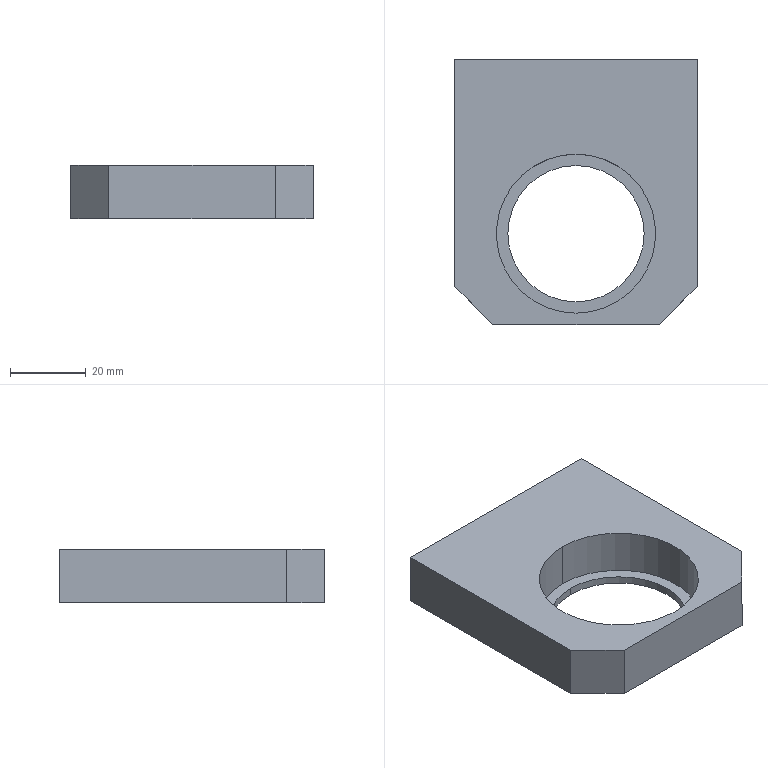Component | SolidWorks | 8TC-A15004-D0-07A-1 | 1 solid | 21 faces | box 64 x 70 x 14 mm | volume 42050 mm3 | plane 9 | cylinder 8 | cone 4 | commonest cylinder face diameters 5 x4 42 x2 36 x2 | material #45
build123d program:
from build123d import *

# Parameters (mm, degrees)
SKETCH1_W             = 64
SKETCH1_H             = 70
BOSS_EXTRUDE1_DEPTH   = 7
SKETCH2_R             = 18
CUT_EXTRUDE1_DEPTH    = 50.447
SKETCH3_R             = 21
CUT_EXTRUDE2_DEPTH    = 12
CHAMFER1_SIZE         = 10
M6_TAPPED_HOLE1_D     = 5
M6_TAPPED_HOLE1_DEPTH = 15
M6_TAPPED_HOLE1_TIP   = 1.502


with BuildPart() as part:
    # Sketch1 → Boss-Extrude1 (new, symmetric)
    with BuildSketch(Plane(origin=(0, 0, 0), x_dir=(1, 0, 0), z_dir=(0, 1, 0))):
        Rectangle(SKETCH1_W, SKETCH1_H)
    extrude(amount=BOSS_EXTRUDE1_DEPTH, both=True)

    # Sketch2 → Cut-Extrude1 (cut, through all)
    with BuildSketch(Plane(origin=(0, 7, 0), x_dir=(1, 0, 0), z_dir=(0, 1, 0))):
        with Locations(Location((0, -11, 0), (0, 0, 270))):
            Circle(SKETCH2_R)
    extrude(amount=-CUT_EXTRUDE1_DEPTH, mode=Mode.SUBTRACT)

    # Sketch3 → Cut-Extrude2 (cut)
    with BuildSketch(Plane(origin=(0, 7, 0), x_dir=(1, 0, 0), z_dir=(0, 1, 0))):
        with Locations(Location((0, -11, 0), (0, 0, 270))):
            Circle(SKETCH3_R)
    extrude(amount=-CUT_EXTRUDE2_DEPTH, mode=Mode.SUBTRACT)

    # Chamfer1
    chamfer1_edges = [part.edges().sort_by_distance(p)[0] for p in [
        (32, 0, 35),
        (-32, 0, 35),
    ]]
    chamfer(chamfer1_edges, length=CHAMFER1_SIZE)

    # M6 Tapped Hole1
    with Locations(Plane(origin=(0, 0, -35), x_dir=(-1, 0, 0), z_dir=(0, 0, -1))):
        with Locations((-25, 0), (25, 0)):
            Hole(M6_TAPPED_HOLE1_D / 2, depth=M6_TAPPED_HOLE1_DEPTH)
            with Locations((0, 0, -(M6_TAPPED_HOLE1_DEPTH + M6_TAPPED_HOLE1_TIP / 2))):  # 118° drill point
                Cone(0, M6_TAPPED_HOLE1_D / 2, M6_TAPPED_HOLE1_TIP, mode=Mode.SUBTRACT)


solid = part.part

# Placed as in the assembly
solid = solid.moved(Location((-7.5, 297.5, -101), (90, 0, 0)))
STEP:
#1=COLOUR_RGB('',0.7922,0.8196,0.9333);
#2=FILL_AREA_STYLE_COLOUR('',#1);
#3=FILL_AREA_STYLE('',(#2));
#4=SURFACE_STYLE_FILL_AREA(#3);
#5=SURFACE_SIDE_STYLE('',(#4));
#6=SURFACE_STYLE_USAGE(.BOTH.,#5);
#7=PRESENTATION_STYLE_ASSIGNMENT((#6));
#8=CARTESIAN_POINT('',(0.7874,12.5,-3.976));
#9=VERTEX_POINT('',#8);
#10=CARTESIAN_POINT('',(0.5906,12.5,-3.976));
#11=VERTEX_POINT('',#10);
#12=CARTESIAN_POINT('',(0.689,12.5,-3.976));
#13=DIRECTION('',(-0.,1.,-0.));
#14=DIRECTION('',(-1.,0.,0.));
#15=AXIS2_PLACEMENT_3D('',#12,#13,#14);
#16=CIRCLE('',#15,0.09843);
#17=EDGE_CURVE('',#9,#11,#16,.T.);
#18=ORIENTED_EDGE('',*,*,#17,.F.);
#19=CARTESIAN_POINT('',(0.7874,13.091,-3.976));
#20=VERTEX_POINT('',#19);
#21=CARTESIAN_POINT('',(0.7874,13.091,-3.976));
#22=DIRECTION('',(-0.,1.,-0.));
#23=VECTOR('',#22,39.37);
#24=LINE('',#21,#23);
#25=EDGE_CURVE('',#9,#20,#24,.T.);
#26=ORIENTED_EDGE('',*,*,#25,.T.);
#27=CARTESIAN_POINT('',(0.5906,13.091,-3.976));
#28=VERTEX_POINT('',#27);
#29=CARTESIAN_POINT('',(0.689,13.091,-3.976));
#30=DIRECTION('',(-0.,1.,-0.));
#31=DIRECTION('',(-1.,0.,0.));
#32=AXIS2_PLACEMENT_3D('',#29,#30,#31);
#33=CIRCLE('',#32,0.09843);
#34=EDGE_CURVE('',#20,#28,#33,.T.);
#35=ORIENTED_EDGE('',*,*,#34,.T.);
#36=CARTESIAN_POINT('',(0.5906,13.091,-3.976));
#37=DIRECTION('',(-0.,1.,-0.));
#38=VECTOR('',#37,39.37);
#39=LINE('',#36,#38);
#40=EDGE_CURVE('',#11,#28,#39,.T.);
#41=ORIENTED_EDGE('',*,*,#40,.F.);
#42=EDGE_LOOP('',(#18,#26,#35,#41));
#43=FACE_OUTER_BOUND('',#42,.T.);
#44=CARTESIAN_POINT('',(0.689,13.091,-3.976));
#45=DIRECTION('',(-0.,1.,-0.));
#46=DIRECTION('',(-1.,0.,0.));
#47=AXIS2_PLACEMENT_3D('',#44,#45,#46);
#48=CYLINDRICAL_SURFACE('',#47,0.09843);
#49=ADVANCED_FACE('',(#43),#48,.F.);
#50=CARTESIAN_POINT('',(0.689,12.441,-3.976));
#51=VERTEX_POINT('',#50);
#52=CARTESIAN_POINT('',(0.5906,12.5,-3.976));
#53=DIRECTION('',(-0.8572,0.515,0.));
#54=VECTOR('',#53,39.37);
#55=LINE('',#52,#54);
#56=EDGE_CURVE('',#51,#11,#55,.T.);
#57=ORIENTED_EDGE('',*,*,#56,.F.);
#58=CARTESIAN_POINT('',(0.7874,12.5,-3.976));
#59=DIRECTION('',(0.8572,0.515,-0.));
#60=VECTOR('',#59,39.37);
#61=LINE('',#58,#60);
#62=EDGE_CURVE('',#51,#9,#61,.T.);
#63=ORIENTED_EDGE('',*,*,#62,.T.);
#64=ORIENTED_EDGE('',*,*,#17,.T.);
#65=EDGE_LOOP('',(#57,#63,#64));
#66=FACE_OUTER_BOUND('',#65,.T.);
#67=CARTESIAN_POINT('',(0.689,12.5,-3.976));
#68=DIRECTION('',(-0.,1.,-0.));
#69=DIRECTION('',(-1.,0.,0.));
#70=AXIS2_PLACEMENT_3D('',#67,#68,#69);
#71=CONICAL_SURFACE('',#70,0.09843,1.03);
#72=ADVANCED_FACE('',(#66),#71,.F.);
#73=CARTESIAN_POINT('',(-1.181,12.5,-3.976));
#74=VERTEX_POINT('',#73);
#75=CARTESIAN_POINT('',(-1.378,12.5,-3.976));
#76=VERTEX_POINT('',#75);
#77=CARTESIAN_POINT('',(-1.28,12.5,-3.976));
#78=DIRECTION('',(-0.,1.,-0.));
#79=DIRECTION('',(-1.,0.,0.));
#80=AXIS2_PLACEMENT_3D('',#77,#78,#79);
#81=CIRCLE('',#80,0.09843);
#82=EDGE_CURVE('',#74,#76,#81,.T.);
#83=ORIENTED_EDGE('',*,*,#82,.F.);
#84=CARTESIAN_POINT('',(-1.181,13.091,-3.976));
#85=VERTEX_POINT('',#84);
#86=CARTESIAN_POINT('',(-1.181,13.091,-3.976));
#87=DIRECTION('',(-0.,1.,-0.));
#88=VECTOR('',#87,39.37);
#89=LINE('',#86,#88);
#90=EDGE_CURVE('',#74,#85,#89,.T.);
#91=ORIENTED_EDGE('',*,*,#90,.T.);
#92=CARTESIAN_POINT('',(-1.378,13.091,-3.976));
#93=VERTEX_POINT('',#92);
#94=CARTESIAN_POINT('',(-1.28,13.091,-3.976));
#95=DIRECTION('',(-0.,1.,-0.));
#96=DIRECTION('',(-1.,0.,0.));
#97=AXIS2_PLACEMENT_3D('',#94,#95,#96);
#98=CIRCLE('',#97,0.09843);
#99=EDGE_CURVE('',#85,#93,#98,.T.);
#100=ORIENTED_EDGE('',*,*,#99,.T.);
#101=CARTESIAN_POINT('',(-1.378,13.091,-3.976));
#102=DIRECTION('',(-0.,1.,-0.));
#103=VECTOR('',#102,39.37);
#104=LINE('',#101,#103);
#105=EDGE_CURVE('',#76,#93,#104,.T.);
#106=ORIENTED_EDGE('',*,*,#105,.F.);
#107=EDGE_LOOP('',(#83,#91,#100,#106));
#108=FACE_OUTER_BOUND('',#107,.T.);
#109=CARTESIAN_POINT('',(-1.28,13.091,-3.976));
#110=DIRECTION('',(-0.,1.,-0.));
#111=DIRECTION('',(-1.,0.,0.));
#112=AXIS2_PLACEMENT_3D('',#109,#110,#111);
#113=CYLINDRICAL_SURFACE('',#112,0.09843);
#114=ADVANCED_FACE('',(#108),#113,.F.);
#115=CARTESIAN_POINT('',(-1.28,12.441,-3.976));
#116=VERTEX_POINT('',#115);
#117=CARTESIAN_POINT('',(-1.378,12.5,-3.976));
#118=DIRECTION('',(-0.8572,0.515,0.));
#119=VECTOR('',#118,39.37);
#120=LINE('',#117,#119);
#121=EDGE_CURVE('',#116,#76,#120,.T.);
#122=ORIENTED_EDGE('',*,*,#121,.F.);
#123=CARTESIAN_POINT('',(-1.181,12.5,-3.976));
#124=DIRECTION('',(0.8572,0.515,-0.));
#125=VECTOR('',#124,39.37);
#126=LINE('',#123,#125);
#127=EDGE_CURVE('',#116,#74,#126,.T.);
#128=ORIENTED_EDGE('',*,*,#127,.T.);
#129=ORIENTED_EDGE('',*,*,#82,.T.);
#130=EDGE_LOOP('',(#122,#128,#129));
#131=FACE_OUTER_BOUND('',#130,.T.);
#132=CARTESIAN_POINT('',(-1.28,12.5,-3.976));
#133=DIRECTION('',(-0.,1.,-0.));
#134=DIRECTION('',(-1.,0.,0.));
#135=AXIS2_PLACEMENT_3D('',#132,#133,#134);
#136=CONICAL_SURFACE('',#135,0.09843,1.03);
#137=ADVANCED_FACE('',(#131),#136,.F.);
#138=CARTESIAN_POINT('',(-0.2953,12.106,-4.173));
#139=VERTEX_POINT('',#138);
#140=CARTESIAN_POINT('',(-0.2953,10.453,-4.173));
#141=VERTEX_POINT('',#140);
#142=CARTESIAN_POINT('',(-0.2953,11.28,-4.173));
#143=DIRECTION('',(0.,0.,1.));
#144=DIRECTION('',(0.,-1.,0.));
#145=AXIS2_PLACEMENT_3D('',#142,#143,#144);
#146=CIRCLE('',#145,0.8268);
#147=EDGE_CURVE('',#139,#141,#146,.T.);
#148=ORIENTED_EDGE('',*,*,#147,.F.);
#149=CARTESIAN_POINT('',(-0.2953,12.106,-3.701));
#150=VERTEX_POINT('',#149);
#151=CARTESIAN_POINT('',(-0.2953,12.106,-4.173));
#152=DIRECTION('',(0.,0.,1.));
#153=VECTOR('',#152,39.37);
#154=LINE('',#151,#153);
#155=EDGE_CURVE('',#139,#150,#154,.T.);
#156=ORIENTED_EDGE('',*,*,#155,.T.);
#157=CARTESIAN_POINT('',(-0.2953,10.453,-3.701));
#158=VERTEX_POINT('',#157);
#159=CARTESIAN_POINT('',(-0.2953,11.28,-3.701));
#160=DIRECTION('',(0.,0.,1.));
#161=DIRECTION('',(0.,-1.,0.));
#162=AXIS2_PLACEMENT_3D('',#159,#160,#161);
#163=CIRCLE('',#162,0.8268);
#164=EDGE_CURVE('',#150,#158,#163,.T.);
#165=ORIENTED_EDGE('',*,*,#164,.T.);
#166=CARTESIAN_POINT('',(-0.2953,10.453,-4.173));
#167=DIRECTION('',(0.,0.,1.));
#168=VECTOR('',#167,39.37);
#169=LINE('',#166,#168);
#170=EDGE_CURVE('',#141,#158,#169,.T.);
#171=ORIENTED_EDGE('',*,*,#170,.F.);
#172=EDGE_LOOP('',(#148,#156,#165,#171));
#173=FACE_OUTER_BOUND('',#172,.T.);
#174=CARTESIAN_POINT('',(-0.2953,11.28,-4.173));
#175=DIRECTION('',(0.,0.,1.));
#176=DIRECTION('',(0.,-1.,0.));
#177=AXIS2_PLACEMENT_3D('',#174,#175,#176);
#178=CYLINDRICAL_SURFACE('',#177,0.8268);
#179=ADVANCED_FACE('',(#173),#178,.F.);
#180=CARTESIAN_POINT('',(-0.2953,11.988,-4.252));
#181=VERTEX_POINT('',#180);
#182=CARTESIAN_POINT('',(-0.2953,10.571,-4.252));
#183=VERTEX_POINT('',#182);
#184=CARTESIAN_POINT('',(-0.2953,11.28,-4.252));
#185=DIRECTION('',(0.,0.,1.));
#186=DIRECTION('',(0.,-1.,0.));
#187=AXIS2_PLACEMENT_3D('',#184,#185,#186);
#188=CIRCLE('',#187,0.7087);
#189=EDGE_CURVE('',#181,#183,#188,.T.);
#190=ORIENTED_EDGE('',*,*,#189,.F.);
#191=CARTESIAN_POINT('',(-0.2953,11.988,-4.173));
#192=VERTEX_POINT('',#191);
#193=CARTESIAN_POINT('',(-0.2953,11.988,-4.252));
#194=DIRECTION('',(0.,0.,1.));
#195=VECTOR('',#194,39.37);
#196=LINE('',#193,#195);
#197=EDGE_CURVE('',#181,#192,#196,.T.);
#198=ORIENTED_EDGE('',*,*,#197,.T.);
#199=CARTESIAN_POINT('',(-0.2953,10.571,-4.173));
#200=VERTEX_POINT('',#199);
#201=CARTESIAN_POINT('',(-0.2953,11.28,-4.173));
#202=DIRECTION('',(-0.,-0.,-1.));
#203=DIRECTION('',(0.,-1.,0.));
#204=AXIS2_PLACEMENT_3D('',#201,#202,#203);
#205=CIRCLE('',#204,0.7087);
#206=EDGE_CURVE('',#200,#192,#205,.T.);
#207=ORIENTED_EDGE('',*,*,#206,.F.);
#208=CARTESIAN_POINT('',(-0.2953,10.571,-4.252));
#209=DIRECTION('',(0.,0.,1.));
#210=VECTOR('',#209,39.37);
#211=LINE('',#208,#210);
#212=EDGE_CURVE('',#183,#200,#211,.T.);
#213=ORIENTED_EDGE('',*,*,#212,.F.);
#214=EDGE_LOOP('',(#190,#198,#207,#213));
#215=FACE_OUTER_BOUND('',#214,.T.);
#216=CARTESIAN_POINT('',(-0.2953,11.28,-4.252));
#217=DIRECTION('',(0.,0.,1.));
#218=DIRECTION('',(0.,-1.,0.));
#219=AXIS2_PLACEMENT_3D('',#216,#217,#218);
#220=CYLINDRICAL_SURFACE('',#219,0.7087);
#221=ADVANCED_FACE('',(#215),#220,.F.);
#222=ORIENTED_EDGE('',*,*,#197,.F.);
#223=CARTESIAN_POINT('',(-0.2953,11.28,-4.252));
#224=DIRECTION('',(0.,0.,1.));
#225=DIRECTION('',(0.,-1.,0.));
#226=AXIS2_PLACEMENT_3D('',#223,#224,#225);
#227=CIRCLE('',#226,0.7087);
#228=EDGE_CURVE('',#183,#181,#227,.T.);
#229=ORIENTED_EDGE('',*,*,#228,.F.);
#230=ORIENTED_EDGE('',*,*,#212,.T.);
#231=CARTESIAN_POINT('',(-0.2953,11.28,-4.173));
#232=DIRECTION('',(-0.,-0.,-1.));
#233=DIRECTION('',(0.,-1.,0.));
#234=AXIS2_PLACEMENT_3D('',#231,#232,#233);
#235=CIRCLE('',#234,0.7087);
#236=EDGE_CURVE('',#192,#200,#235,.T.);
#237=ORIENTED_EDGE('',*,*,#236,.F.);
#238=EDGE_LOOP('',(#222,#229,#230,#237));
#239=FACE_OUTER_BOUND('',#238,.T.);
#240=CARTESIAN_POINT('',(-0.2953,11.28,-4.252));
#241=DIRECTION('',(0.,0.,1.));
#242=DIRECTION('',(0.,-1.,0.));
#243=AXIS2_PLACEMENT_3D('',#240,#241,#242);
#244=CYLINDRICAL_SURFACE('',#243,0.7087);
#245=ADVANCED_FACE('',(#239),#244,.F.);
#246=CARTESIAN_POINT('',(0.9646,10.728,-3.701));
#247=VERTEX_POINT('',#246);
#248=CARTESIAN_POINT('',(0.9646,13.091,-3.701));
#249=VERTEX_POINT('',#248);
#250=CARTESIAN_POINT('',(0.9646,10.335,-3.701));
#251=DIRECTION('',(-0.,1.,-0.));
#252=VECTOR('',#251,39.37);
#253=LINE('',#250,#252);
#254=EDGE_CURVE('',#247,#249,#253,.T.);
#255=ORIENTED_EDGE('',*,*,#254,.F.);
#256=CARTESIAN_POINT('',(0.9646,10.728,-4.252));
#257=VERTEX_POINT('',#256);
#258=CARTESIAN_POINT('',(0.9646,10.728,-3.701));
#259=DIRECTION('',(-0.,-0.,-1.));
#260=VECTOR('',#259,39.37);
#261=LINE('',#258,#260);
#262=EDGE_CURVE('',#247,#257,#261,.T.);
#263=ORIENTED_EDGE('',*,*,#262,.T.);
#264=CARTESIAN_POINT('',(0.9646,13.091,-4.252));
#265=VERTEX_POINT('',#264);
#266=CARTESIAN_POINT('',(0.9646,10.335,-4.252));
#267=DIRECTION('',(-0.,1.,-0.));
#268=VECTOR('',#267,39.37);
#269=LINE('',#266,#268);
#270=EDGE_CURVE('',#257,#265,#269,.T.);
#271=ORIENTED_EDGE('',*,*,#270,.T.);
#272=CARTESIAN_POINT('',(0.9646,13.091,-3.701));
#273=DIRECTION('',(-0.,-0.,-1.));
#274=VECTOR('',#273,39.37);
#275=LINE('',#272,#274);
#276=EDGE_CURVE('',#249,#265,#275,.T.);
#277=ORIENTED_EDGE('',*,*,#276,.F.);
#278=EDGE_LOOP('',(#255,#263,#271,#277));
#279=FACE_OUTER_BOUND('',#278,.T.);
#280=CARTESIAN_POINT('',(0.9646,10.335,-3.701));
#281=DIRECTION('',(-1.,-0.,0.));
#282=DIRECTION('',(0.,-1.,0.));
#283=AXIS2_PLACEMENT_3D('',#280,#281,#282);
#284=PLANE('',#283);
#285=ADVANCED_FACE('',(#279),#284,.F.);
#286=CARTESIAN_POINT('',(0.689,13.091,-3.976));
#287=DIRECTION('',(-0.,1.,-0.));
#288=DIRECTION('',(-1.,0.,0.));
#289=AXIS2_PLACEMENT_3D('',#286,#287,#288);
#290=CIRCLE('',#289,0.09843);
#291=EDGE_CURVE('',#28,#20,#290,.T.);
#292=ORIENTED_EDGE('',*,*,#291,.F.);
#293=ORIENTED_EDGE('',*,*,#34,.F.);
#294=EDGE_LOOP('',(#292,#293));
#295=FACE_BOUND('',#294,.T.);
#296=CARTESIAN_POINT('',(-1.28,13.091,-3.976));
#297=DIRECTION('',(-0.,1.,-0.));
#298=DIRECTION('',(-1.,0.,0.));
#299=AXIS2_PLACEMENT_3D('',#296,#297,#298);
#300=CIRCLE('',#299,0.09843);
#301=EDGE_CURVE('',#93,#85,#300,.T.);
#302=ORIENTED_EDGE('',*,*,#301,.F.);
#303=ORIENTED_EDGE('',*,*,#99,.F.);
#304=EDGE_LOOP('',(#302,#303));
#305=FACE_BOUND('',#304,.T.);
#306=CARTESIAN_POINT('',(-1.555,13.091,-4.252));
#307=VERTEX_POINT('',#306);
#308=CARTESIAN_POINT('',(-1.555,13.091,-4.252));
#309=DIRECTION('',(-1.,-0.,0.));
#310=VECTOR('',#309,39.37);
#311=LINE('',#308,#310);
#312=EDGE_CURVE('',#265,#307,#311,.T.);
#313=ORIENTED_EDGE('',*,*,#312,.T.);
#314=CARTESIAN_POINT('',(-1.555,13.091,-3.701));
#315=VERTEX_POINT('',#314);
#316=CARTESIAN_POINT('',(-1.555,13.091,-3.701));
#317=DIRECTION('',(-0.,-0.,-1.));
#318=VECTOR('',#317,39.37);
#319=LINE('',#316,#318);
#320=EDGE_CURVE('',#315,#307,#319,.T.);
#321=ORIENTED_EDGE('',*,*,#320,.F.);
#322=CARTESIAN_POINT('',(-1.555,13.091,-3.701));
#323=DIRECTION('',(-1.,-0.,0.));
#324=VECTOR('',#323,39.37);
#325=LINE('',#322,#324);
#326=EDGE_CURVE('',#249,#315,#325,.T.);
#327=ORIENTED_EDGE('',*,*,#326,.F.);
#328=ORIENTED_EDGE('',*,*,#276,.T.);
#329=EDGE_LOOP('',(#313,#321,#327,#328));
#330=FACE_OUTER_BOUND('',#329,.T.);
#331=CARTESIAN_POINT('',(-1.555,13.091,-3.701));
#332=DIRECTION('',(0.,-1.,0.));
#333=DIRECTION('',(1.,0.,-0.));
#334=AXIS2_PLACEMENT_3D('',#331,#332,#333);
#335=PLANE('',#334);
#336=ADVANCED_FACE('',(#295,#305,#330),#335,.F.);
#337=CARTESIAN_POINT('',(-1.555,10.728,-4.252));
#338=VERTEX_POINT('',#337);
#339=CARTESIAN_POINT('',(-1.555,10.335,-4.252));
#340=DIRECTION('',(0.,-1.,0.));
#341=VECTOR('',#340,39.37);
#342=LINE('',#339,#341);
#343=EDGE_CURVE('',#307,#338,#342,.T.);
#344=ORIENTED_EDGE('',*,*,#343,.T.);
#345=CARTESIAN_POINT('',(-1.555,10.728,-3.701));
#346=VERTEX_POINT('',#345);
#347=CARTESIAN_POINT('',(-1.555,10.728,-3.701));
#348=DIRECTION('',(0.,0.,1.));
#349=VECTOR('',#348,39.37);
#350=LINE('',#347,#349);
#351=EDGE_CURVE('',#338,#346,#350,.T.);
#352=ORIENTED_EDGE('',*,*,#351,.T.);
#353=CARTESIAN_POINT('',(-1.555,10.335,-3.701));
#354=DIRECTION('',(0.,-1.,0.));
#355=VECTOR('',#354,39.37);
#356=LINE('',#353,#355);
#357=EDGE_CURVE('',#315,#346,#356,.T.);
#358=ORIENTED_EDGE('',*,*,#357,.F.);
#359=ORIENTED_EDGE('',*,*,#320,.T.);
#360=EDGE_LOOP('',(#344,#352,#358,#359));
#361=FACE_OUTER_BOUND('',#360,.T.);
#362=CARTESIAN_POINT('',(-1.555,10.335,-3.701));
#363=DIRECTION('',(1.,0.,-0.));
#364=DIRECTION('',(-0.,1.,-0.));
#365=AXIS2_PLACEMENT_3D('',#362,#363,#364);
#366=PLANE('',#365);
#367=ADVANCED_FACE('',(#361),#366,.F.);
#368=CARTESIAN_POINT('',(-1.161,10.335,-3.701));
#369=VERTEX_POINT('',#368);
#370=CARTESIAN_POINT('',(0.5709,10.335,-3.701));
#371=VERTEX_POINT('',#370);
#372=CARTESIAN_POINT('',(-1.555,10.335,-3.701));
#373=DIRECTION('',(1.,0.,-0.));
#374=VECTOR('',#373,39.37);
#375=LINE('',#372,#374);
#376=EDGE_CURVE('',#369,#371,#375,.T.);
#377=ORIENTED_EDGE('',*,*,#376,.F.);
#378=CARTESIAN_POINT('',(-1.161,10.335,-4.252));
#379=VERTEX_POINT('',#378);
#380=CARTESIAN_POINT('',(-1.161,10.335,-3.701));
#381=DIRECTION('',(-0.,-0.,-1.));
#382=VECTOR('',#381,39.37);
#383=LINE('',#380,#382);
#384=EDGE_CURVE('',#369,#379,#383,.T.);
#385=ORIENTED_EDGE('',*,*,#384,.T.);
#386=CARTESIAN_POINT('',(0.5709,10.335,-4.252));
#387=VERTEX_POINT('',#386);
#388=CARTESIAN_POINT('',(-1.555,10.335,-4.252));
#389=DIRECTION('',(1.,0.,-0.));
#390=VECTOR('',#389,39.37);
#391=LINE('',#388,#390);
#392=EDGE_CURVE('',#379,#387,#391,.T.);
#393=ORIENTED_EDGE('',*,*,#392,.T.);
#394=CARTESIAN_POINT('',(0.5709,10.335,-3.701));
#395=DIRECTION('',(0.,0.,1.));
#396=VECTOR('',#395,39.37);
#397=LINE('',#394,#396);
#398=EDGE_CURVE('',#387,#371,#397,.T.);
#399=ORIENTED_EDGE('',*,*,#398,.T.);
#400=EDGE_LOOP('',(#377,#385,#393,#399));
#401=FACE_OUTER_BOUND('',#400,.T.);
#402=CARTESIAN_POINT('',(-1.555,10.335,-3.701));
#403=DIRECTION('',(-0.,1.,-0.));
#404=DIRECTION('',(-1.,-0.,0.));
#405=AXIS2_PLACEMENT_3D('',#402,#403,#404);
#406=PLANE('',#405);
#407=ADVANCED_FACE('',(#401),#406,.F.);
#408=CARTESIAN_POINT('',(-0.2953,11.28,-3.701));
#409=DIRECTION('',(0.,0.,1.));
#410=DIRECTION('',(0.,-1.,0.));
#411=AXIS2_PLACEMENT_3D('',#408,#409,#410);
#412=CIRCLE('',#411,0.8268);
#413=EDGE_CURVE('',#158,#150,#412,.T.);
#414=ORIENTED_EDGE('',*,*,#413,.F.);
#415=ORIENTED_EDGE('',*,*,#164,.F.);
#416=EDGE_LOOP('',(#414,#415));
#417=FACE_BOUND('',#416,.T.);
#418=ORIENTED_EDGE('',*,*,#357,.T.);
#419=CARTESIAN_POINT('',(-1.161,10.335,-3.701));
#420=DIRECTION('',(0.7071,-0.7071,-0.));
#421=VECTOR('',#420,39.37);
#422=LINE('',#419,#421);
#423=EDGE_CURVE('',#346,#369,#422,.T.);
#424=ORIENTED_EDGE('',*,*,#423,.T.);
#425=ORIENTED_EDGE('',*,*,#376,.T.);
#426=CARTESIAN_POINT('',(0.9646,10.728,-3.701));
#427=DIRECTION('',(0.7071,0.7071,-0.));
#428=VECTOR('',#427,39.37);
#429=LINE('',#426,#428);
#430=EDGE_CURVE('',#371,#247,#429,.T.);
#431=ORIENTED_EDGE('',*,*,#430,.T.);
#432=ORIENTED_EDGE('',*,*,#254,.T.);
#433=ORIENTED_EDGE('',*,*,#326,.T.);
#434=EDGE_LOOP('',(#418,#424,#425,#431,#432,#433));
#435=FACE_OUTER_BOUND('',#434,.T.);
#436=CARTESIAN_POINT('',(-0.2953,11.713,-3.701));
#437=DIRECTION('',(-0.,-0.,-1.));
#438=DIRECTION('',(-0.,1.,-0.));
#439=AXIS2_PLACEMENT_3D('',#436,#437,#438);
#440=PLANE('',#439);
#441=ADVANCED_FACE('',(#417,#435),#440,.F.);
#442=ORIENTED_EDGE('',*,*,#228,.T.);
#443=ORIENTED_EDGE('',*,*,#189,.T.);
#444=EDGE_LOOP('',(#442,#443));
#445=FACE_BOUND('',#444,.T.);
#446=ORIENTED_EDGE('',*,*,#392,.F.);
#447=CARTESIAN_POINT('',(-1.417,10.591,-4.252));
#448=DIRECTION('',(-0.7071,0.7071,0.));
#449=VECTOR('',#448,39.37);
#450=LINE('',#447,#449);
#451=EDGE_CURVE('',#379,#338,#450,.T.);
#452=ORIENTED_EDGE('',*,*,#451,.T.);
#453=ORIENTED_EDGE('',*,*,#343,.F.);
#454=ORIENTED_EDGE('',*,*,#312,.F.);
#455=ORIENTED_EDGE('',*,*,#270,.F.);
#456=CARTESIAN_POINT('',(0.8268,10.591,-4.252));
#457=DIRECTION('',(-0.7071,-0.7071,0.));
#458=VECTOR('',#457,39.37);
#459=LINE('',#456,#458);
#460=EDGE_CURVE('',#257,#387,#459,.T.);
#461=ORIENTED_EDGE('',*,*,#460,.T.);
#462=EDGE_LOOP('',(#446,#452,#453,#454,#455,#461));
#463=FACE_OUTER_BOUND('',#462,.T.);
#464=CARTESIAN_POINT('',(-0.2953,11.713,-4.252));
#465=DIRECTION('',(-0.,-0.,-1.));
#466=DIRECTION('',(-0.,1.,-0.));
#467=AXIS2_PLACEMENT_3D('',#464,#465,#466);
#468=PLANE('',#467);
#469=ADVANCED_FACE('',(#445,#463),#468,.T.);
#470=CARTESIAN_POINT('',(-0.2953,11.28,-4.173));
#471=DIRECTION('',(0.,0.,1.));
#472=DIRECTION('',(0.,-1.,0.));
#473=AXIS2_PLACEMENT_3D('',#470,#471,#472);
#474=CIRCLE('',#473,0.8268);
#475=EDGE_CURVE('',#141,#139,#474,.T.);
#476=ORIENTED_EDGE('',*,*,#475,.T.);
#477=ORIENTED_EDGE('',*,*,#147,.T.);
#478=EDGE_LOOP('',(#476,#477));
#479=FACE_OUTER_BOUND('',#478,.T.);
#480=ORIENTED_EDGE('',*,*,#206,.T.);
#481=ORIENTED_EDGE('',*,*,#236,.T.);
#482=EDGE_LOOP('',(#480,#481));
#483=FACE_BOUND('',#482,.T.);
#484=CARTESIAN_POINT('',(-0.2953,11.28,-4.173));
#485=DIRECTION('',(0.,0.,1.));
#486=DIRECTION('',(0.,-1.,0.));
#487=AXIS2_PLACEMENT_3D('',#484,#485,#486);
#488=PLANE('',#487);
#489=ADVANCED_FACE('',(#479,#483),#488,.T.);
#490=ORIENTED_EDGE('',*,*,#155,.F.);
#491=ORIENTED_EDGE('',*,*,#475,.F.);
#492=ORIENTED_EDGE('',*,*,#170,.T.);
#493=ORIENTED_EDGE('',*,*,#413,.T.);
#494=EDGE_LOOP('',(#490,#491,#492,#493));
#495=FACE_OUTER_BOUND('',#494,.T.);
#496=CARTESIAN_POINT('',(-0.2953,11.28,-4.173));
#497=DIRECTION('',(0.,0.,1.));
#498=DIRECTION('',(0.,-1.,0.));
#499=AXIS2_PLACEMENT_3D('',#496,#497,#498);
#500=CYLINDRICAL_SURFACE('',#499,0.8268);
#501=ADVANCED_FACE('',(#495),#500,.F.);
#502=ORIENTED_EDGE('',*,*,#423,.F.);
#503=ORIENTED_EDGE('',*,*,#351,.F.);
#504=ORIENTED_EDGE('',*,*,#451,.F.);
#505=ORIENTED_EDGE('',*,*,#384,.F.);
#506=EDGE_LOOP('',(#502,#503,#504,#505));
#507=FACE_OUTER_BOUND('',#506,.T.);
#508=CARTESIAN_POINT('',(-1.161,10.335,-3.701));
#509=DIRECTION('',(0.7071,0.7071,-0.));
#510=DIRECTION('',(-0.,-0.,-1.));
#511=AXIS2_PLACEMENT_3D('',#508,#509,#510);
#512=PLANE('',#511);
#513=ADVANCED_FACE('',(#507),#512,.F.);
#514=ORIENTED_EDGE('',*,*,#430,.F.);
#515=ORIENTED_EDGE('',*,*,#398,.F.);
#516=ORIENTED_EDGE('',*,*,#460,.F.);
#517=ORIENTED_EDGE('',*,*,#262,.F.);
#518=EDGE_LOOP('',(#514,#515,#516,#517));
#519=FACE_OUTER_BOUND('',#518,.T.);
#520=CARTESIAN_POINT('',(0.9646,10.728,-3.701));
#521=DIRECTION('',(-0.7071,0.7071,0.));
#522=DIRECTION('',(-0.,-0.,-1.));
#523=AXIS2_PLACEMENT_3D('',#520,#521,#522);
#524=PLANE('',#523);
#525=ADVANCED_FACE('',(#519),#524,.F.);
#526=ORIENTED_EDGE('',*,*,#127,.F.);
#527=ORIENTED_EDGE('',*,*,#121,.T.);
#528=CARTESIAN_POINT('',(-1.28,12.5,-3.976));
#529=DIRECTION('',(-0.,1.,-0.));
#530=DIRECTION('',(-1.,0.,0.));
#531=AXIS2_PLACEMENT_3D('',#528,#529,#530);
#532=CIRCLE('',#531,0.09843);
#533=EDGE_CURVE('',#76,#74,#532,.T.);
#534=ORIENTED_EDGE('',*,*,#533,.T.);
#535=EDGE_LOOP('',(#526,#527,#534));
#536=FACE_OUTER_BOUND('',#535,.T.);
#537=CARTESIAN_POINT('',(-1.28,12.5,-3.976));
#538=DIRECTION('',(-0.,1.,-0.));
#539=DIRECTION('',(-1.,0.,0.));
#540=AXIS2_PLACEMENT_3D('',#537,#538,#539);
#541=CONICAL_SURFACE('',#540,0.09843,1.03);
#542=ADVANCED_FACE('',(#536),#541,.F.);
#543=ORIENTED_EDGE('',*,*,#90,.F.);
#544=ORIENTED_EDGE('',*,*,#533,.F.);
#545=ORIENTED_EDGE('',*,*,#105,.T.);
#546=ORIENTED_EDGE('',*,*,#301,.T.);
#547=EDGE_LOOP('',(#543,#544,#545,#546));
#548=FACE_OUTER_BOUND('',#547,.T.);
#549=CARTESIAN_POINT('',(-1.28,13.091,-3.976));
#550=DIRECTION('',(-0.,1.,-0.));
#551=DIRECTION('',(-1.,0.,0.));
#552=AXIS2_PLACEMENT_3D('',#549,#550,#551);
#553=CYLINDRICAL_SURFACE('',#552,0.09843);
#554=ADVANCED_FACE('',(#548),#553,.F.);
#555=ORIENTED_EDGE('',*,*,#62,.F.);
#556=ORIENTED_EDGE('',*,*,#56,.T.);
#557=CARTESIAN_POINT('',(0.689,12.5,-3.976));
#558=DIRECTION('',(-0.,1.,-0.));
#559=DIRECTION('',(-1.,0.,0.));
#560=AXIS2_PLACEMENT_3D('',#557,#558,#559);
#561=CIRCLE('',#560,0.09843);
#562=EDGE_CURVE('',#11,#9,#561,.T.);
#563=ORIENTED_EDGE('',*,*,#562,.T.);
#564=EDGE_LOOP('',(#555,#556,#563));
#565=FACE_OUTER_BOUND('',#564,.T.);
#566=CARTESIAN_POINT('',(0.689,12.5,-3.976));
#567=DIRECTION('',(-0.,1.,-0.));
#568=DIRECTION('',(-1.,0.,0.));
#569=AXIS2_PLACEMENT_3D('',#566,#567,#568);
#570=CONICAL_SURFACE('',#569,0.09843,1.03);
#571=ADVANCED_FACE('',(#565),#570,.F.);
#572=ORIENTED_EDGE('',*,*,#25,.F.);
#573=ORIENTED_EDGE('',*,*,#562,.F.);
#574=ORIENTED_EDGE('',*,*,#40,.T.);
#575=ORIENTED_EDGE('',*,*,#291,.T.);
#576=EDGE_LOOP('',(#572,#573,#574,#575));
#577=FACE_OUTER_BOUND('',#576,.T.);
#578=CARTESIAN_POINT('',(0.689,13.091,-3.976));
#579=DIRECTION('',(-0.,1.,-0.));
#580=DIRECTION('',(-1.,0.,0.));
#581=AXIS2_PLACEMENT_3D('',#578,#579,#580);
#582=CYLINDRICAL_SURFACE('',#581,0.09843);
#583=ADVANCED_FACE('',(#577),#582,.F.);
#584=CLOSED_SHELL('',(#49,#72,#114,#137,#179,#221,#245,#285,#336,#367,#407,#441,#469,#489,#501,#513,#525,#542,#554,#571,#583));
#585=MANIFOLD_SOLID_BREP('',#584);
#586=STYLED_ITEM('',(#7),#585);
#587=PRESENTATION_LAYER_ASSIGNMENT('','',(#586));
#588=CARTESIAN_POINT('',(0.,0.,0.));
#589=DIRECTION('',(0.,0.,1.));
#590=DIRECTION('',(1.,0.,0.));
#591=AXIS2_PLACEMENT_3D('',#588,#589,#590);
#592=(LENGTH_UNIT()NAMED_UNIT(*)SI_UNIT($,.METRE.));
#593=LENGTH_MEASURE_WITH_UNIT(LENGTH_MEASURE(0.0254),#592);
#594=DIMENSIONAL_EXPONENTS(1.,0.,0.,0.,0.,0.,0.);
#595=(CONVERSION_BASED_UNIT('',#593)LENGTH_UNIT()NAMED_UNIT(#594));
#596=UNCERTAINTY_MEASURE_WITH_UNIT(LENGTH_MEASURE(0.00001),#595,'','');
#597=(NAMED_UNIT(*)PLANE_ANGLE_UNIT()SI_UNIT($,.RADIAN.));
#598=(NAMED_UNIT(*)SI_UNIT($,.STERADIAN.)SOLID_ANGLE_UNIT());
#599=(GEOMETRIC_REPRESENTATION_CONTEXT(3)GLOBAL_UNCERTAINTY_ASSIGNED_CONTEXT((#596))GLOBAL_UNIT_ASSIGNED_CONTEXT((#595,#597,#598))REPRESENTATION_CONTEXT('',''));
#600=ADVANCED_BREP_SHAPE_REPRESENTATION('',(#585,#591),#599);
#601=(LENGTH_UNIT()NAMED_UNIT(*)SI_UNIT($,.METRE.));
#602=LENGTH_MEASURE_WITH_UNIT(LENGTH_MEASURE(0.0254),#601);
#603=DIMENSIONAL_EXPONENTS(1.,0.,0.,0.,0.,0.,0.);
#604=(CONVERSION_BASED_UNIT('',#602)LENGTH_UNIT()NAMED_UNIT(#603));
#605=UNCERTAINTY_MEASURE_WITH_UNIT(LENGTH_MEASURE(0.00001),#604,'','');
#606=(NAMED_UNIT(*)PLANE_ANGLE_UNIT()SI_UNIT($,.RADIAN.));
#607=(NAMED_UNIT(*)SI_UNIT($,.STERADIAN.)SOLID_ANGLE_UNIT());
#608=(GEOMETRIC_REPRESENTATION_CONTEXT(3)GLOBAL_UNCERTAINTY_ASSIGNED_CONTEXT((#605))GLOBAL_UNIT_ASSIGNED_CONTEXT((#604,#606,#607))REPRESENTATION_CONTEXT('',''));
#609=MECHANICAL_DESIGN_GEOMETRIC_PRESENTATION_REPRESENTATION('',(#586),#608);